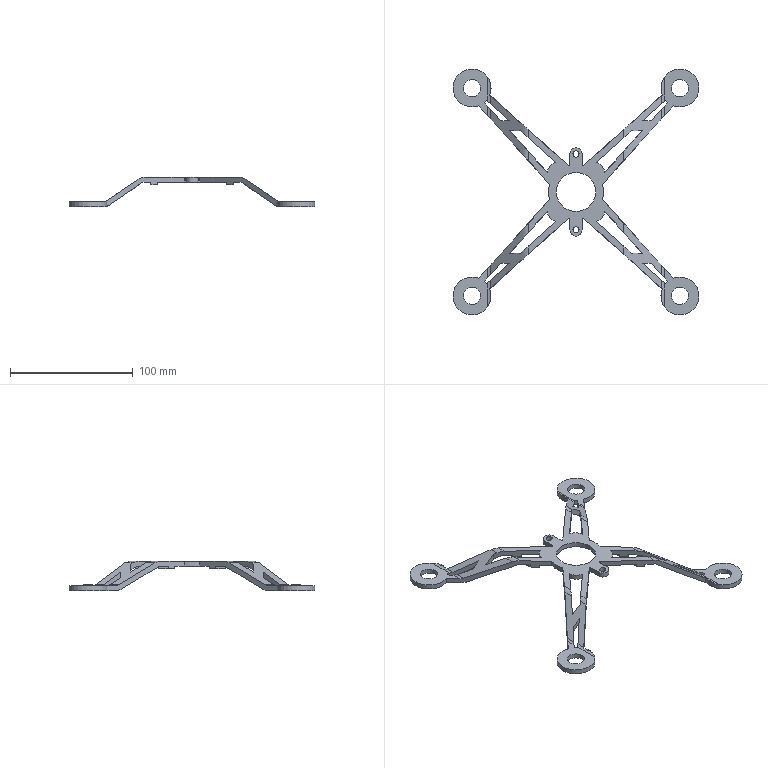Component | NX | BRACKET | 1 solid | 141 faces | volume 31493 mm3 | plane 90 | cylinder 51 | commonest cylinder face diameters 16 x16 8 x8 31 x8 45 x6 14 x4 20 x4 10 x2 5 x2